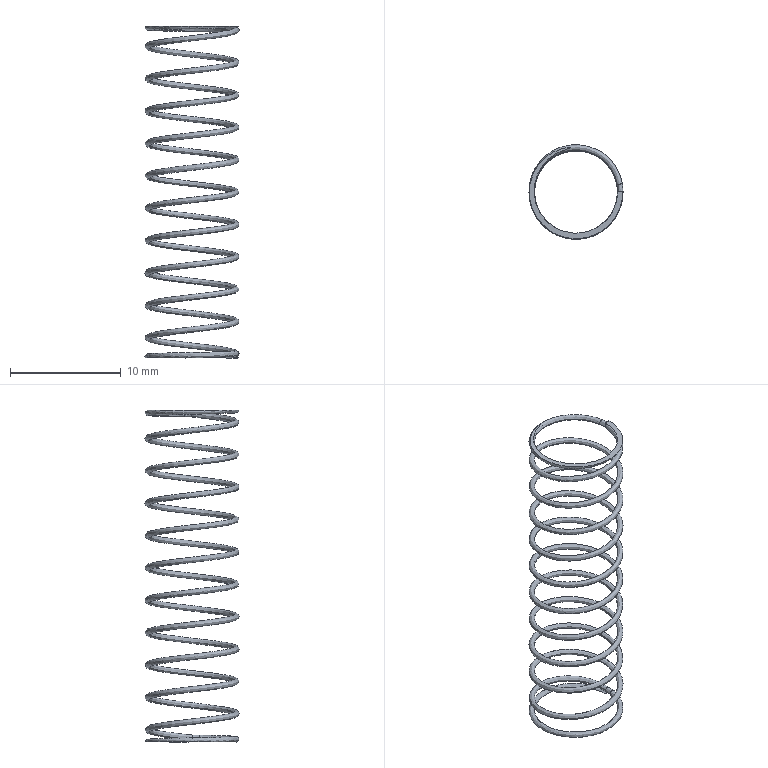Component | NX | SPRING | 1 solid | 9 faces | volume 60 mm3 | spline 5 | plane 4